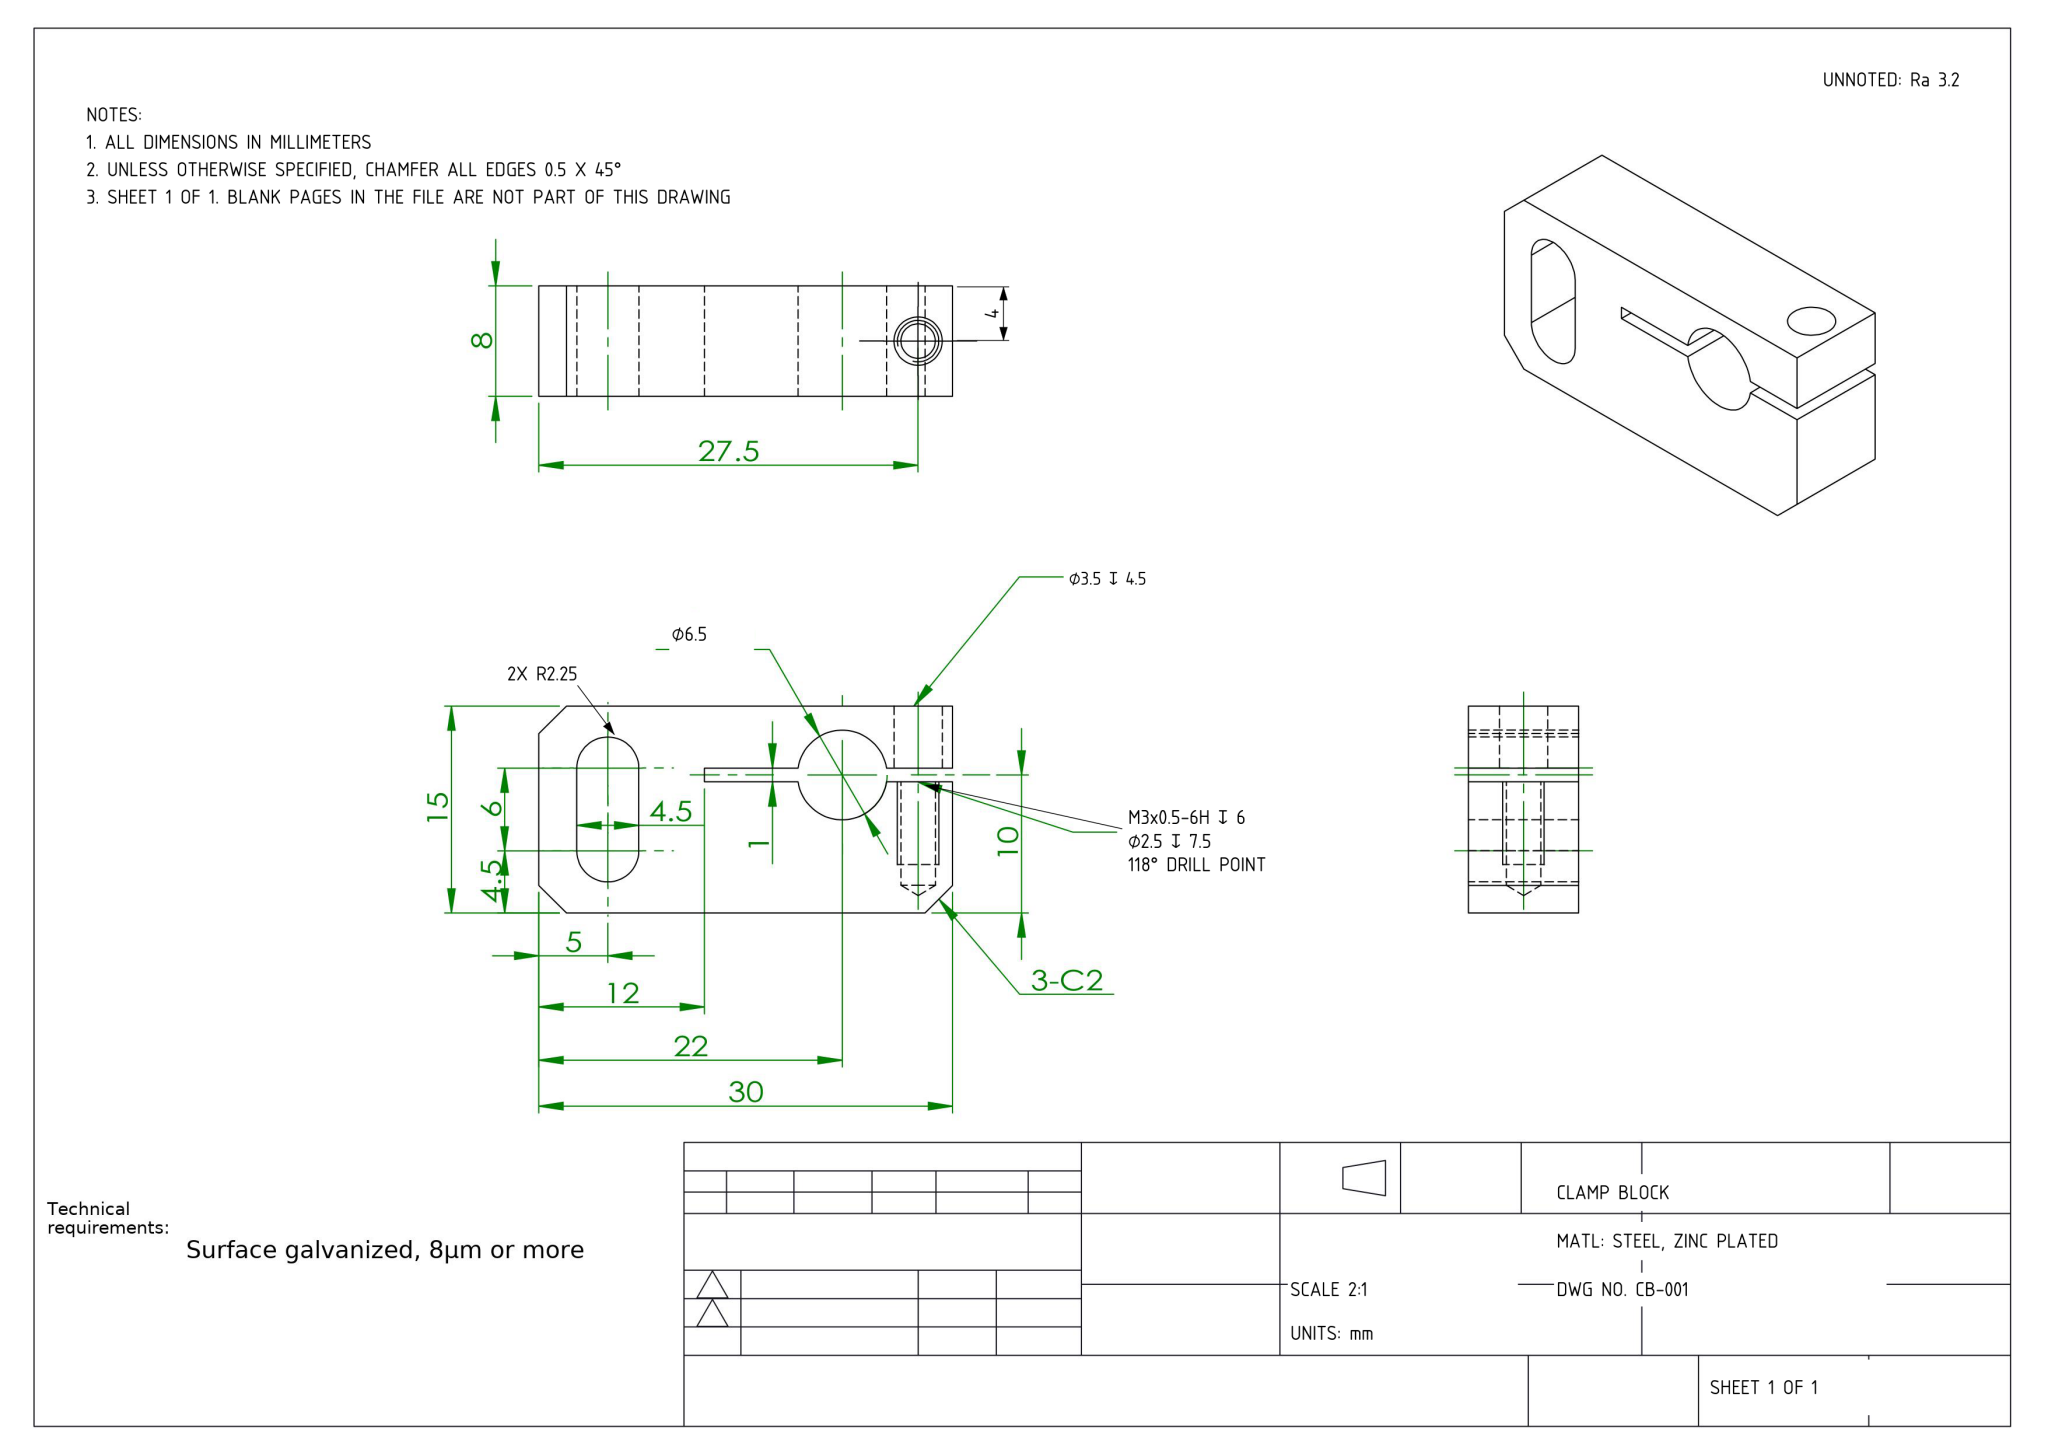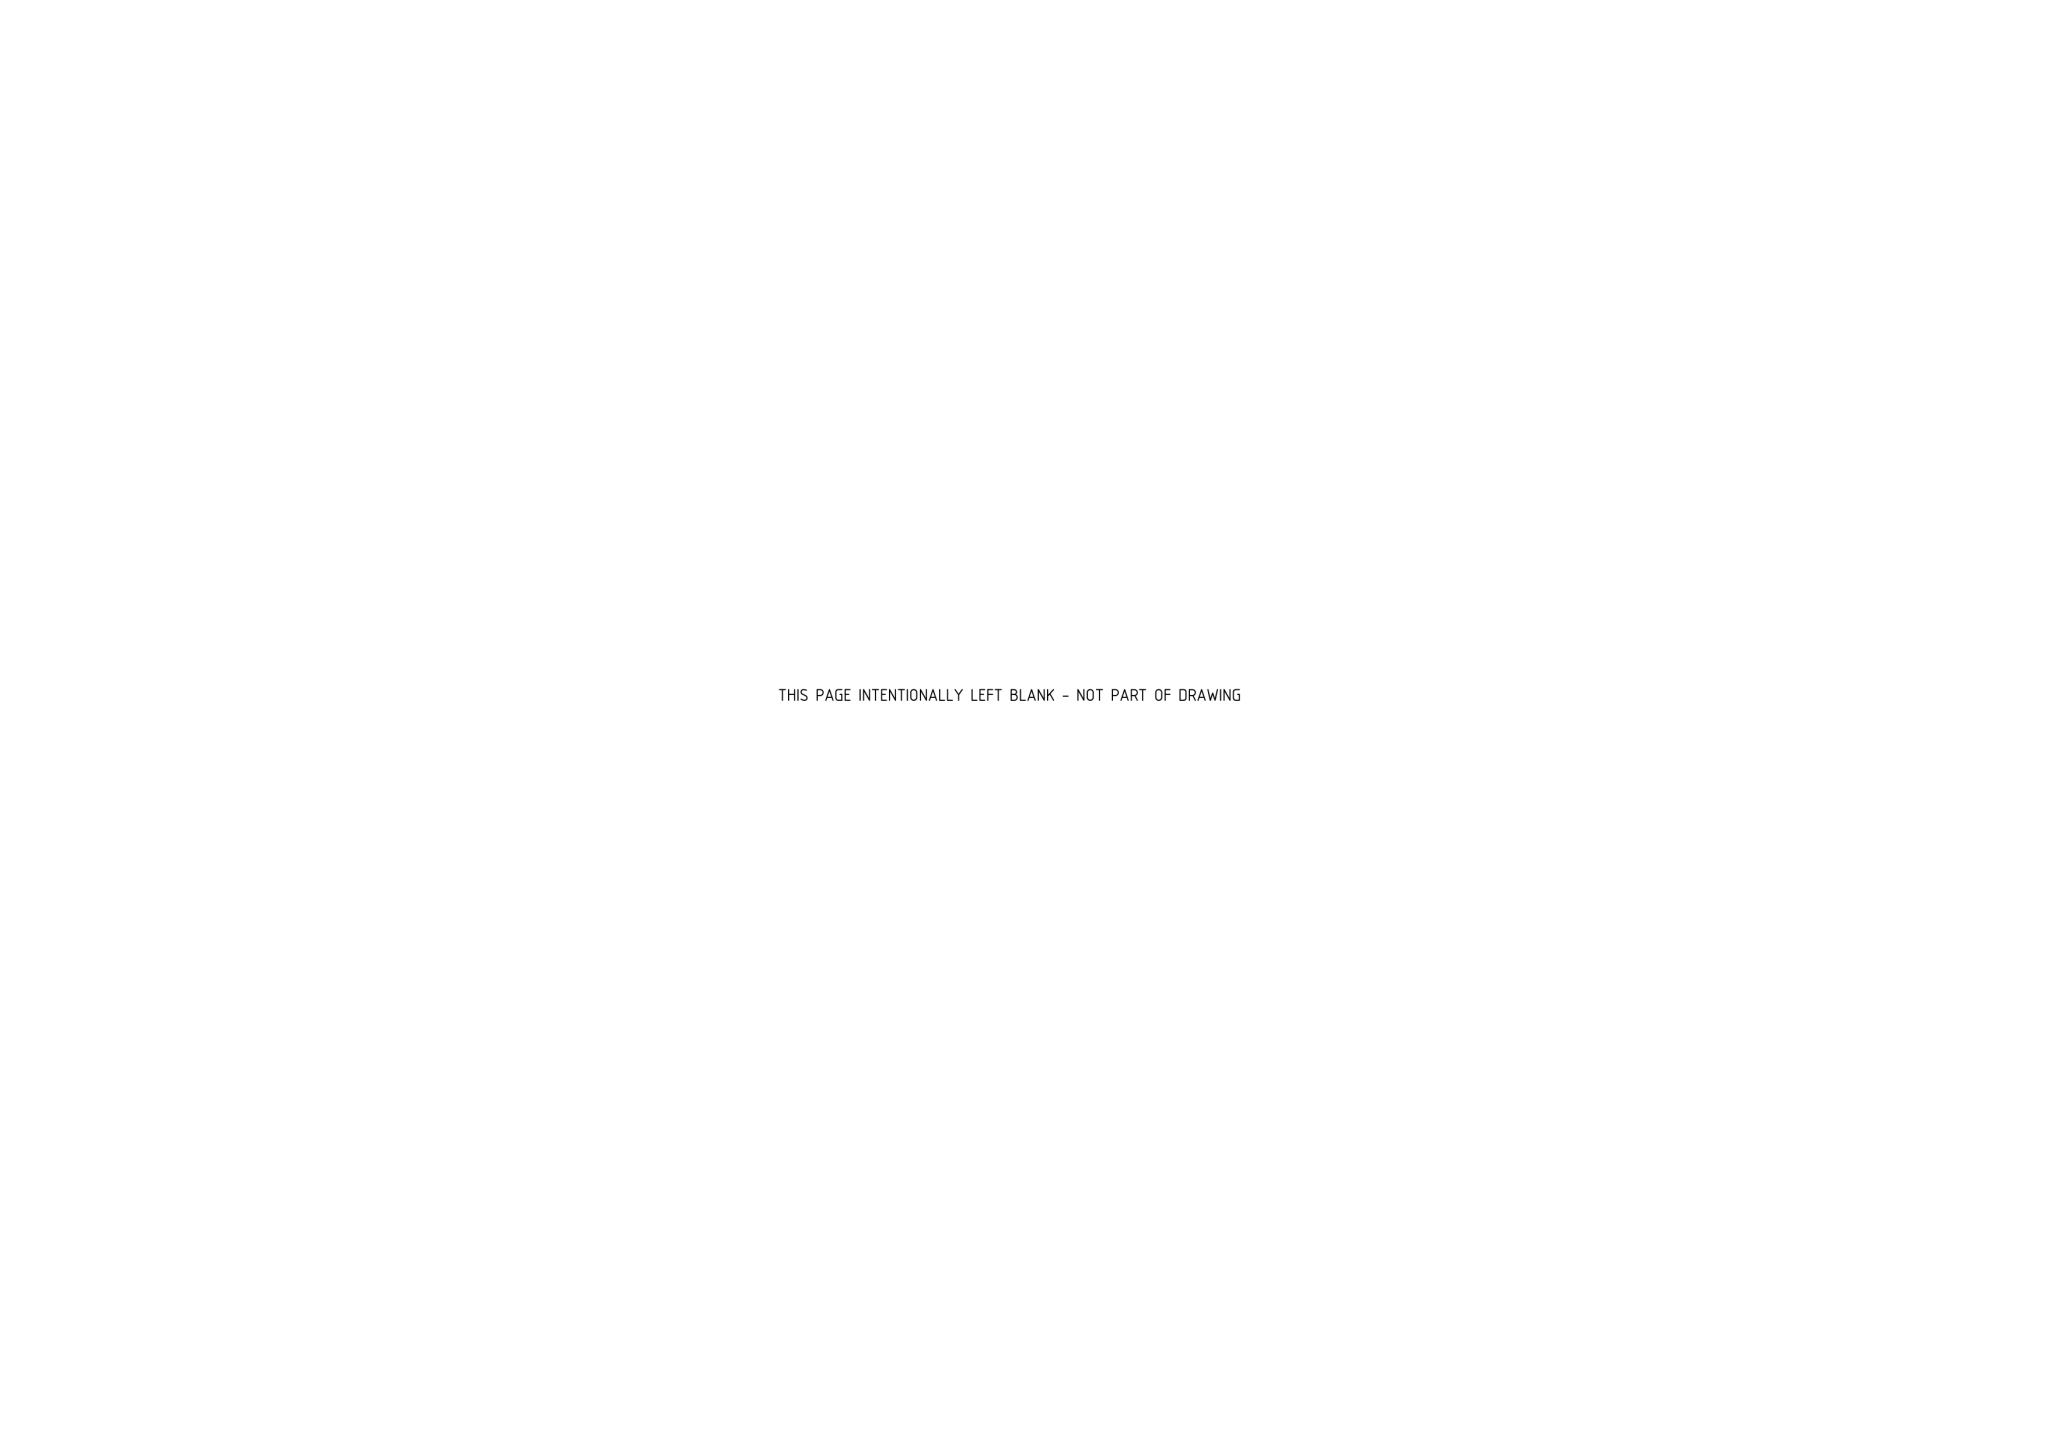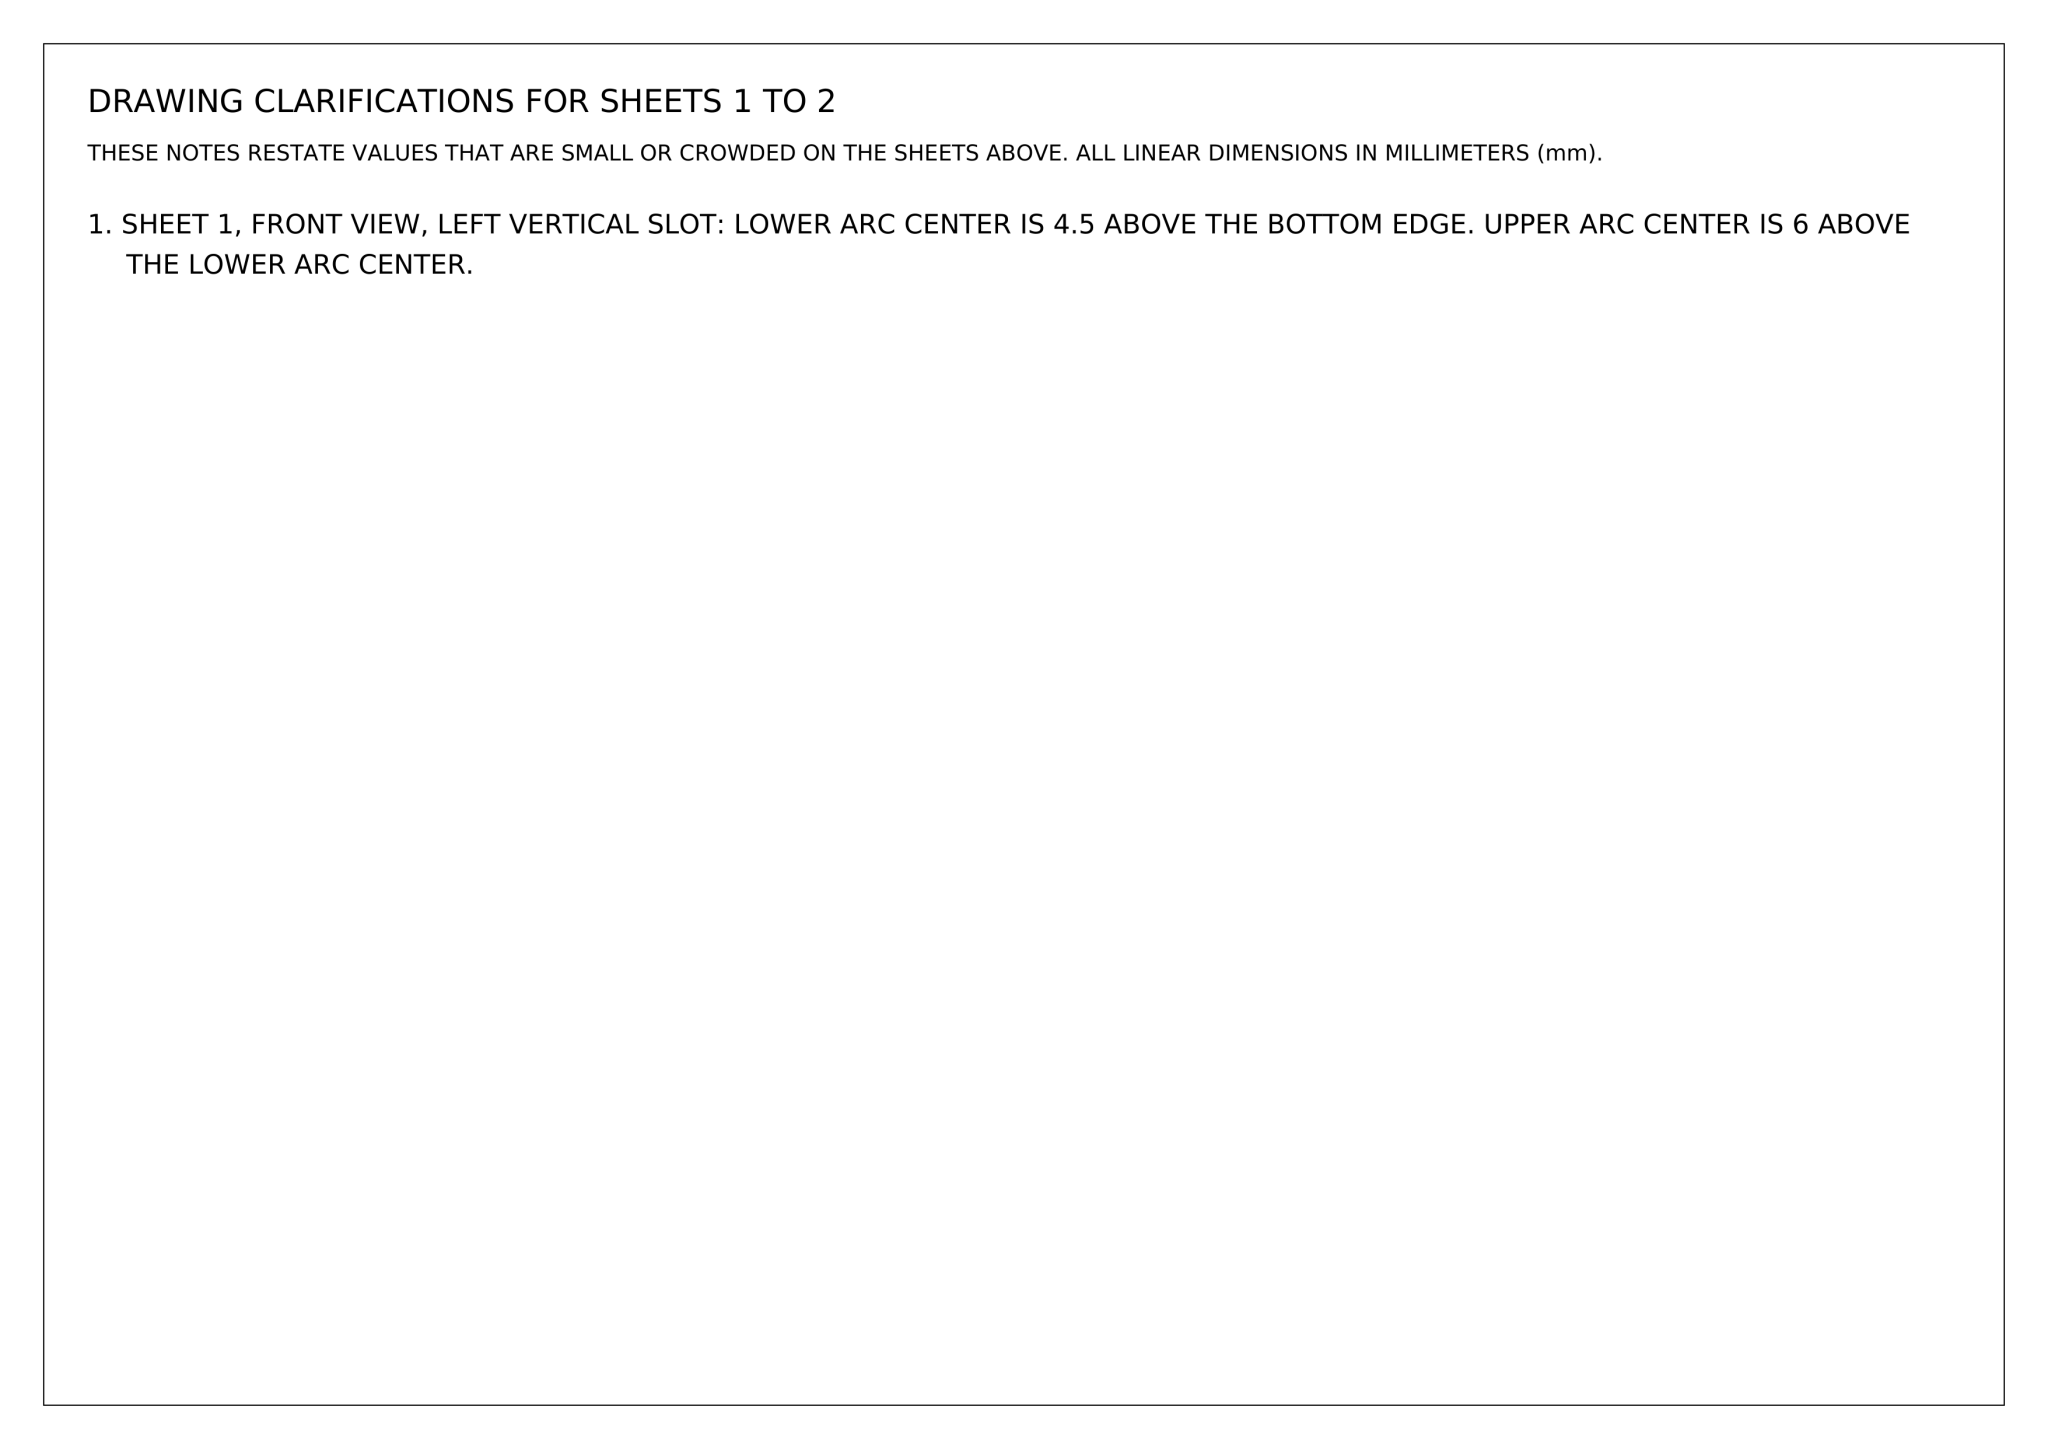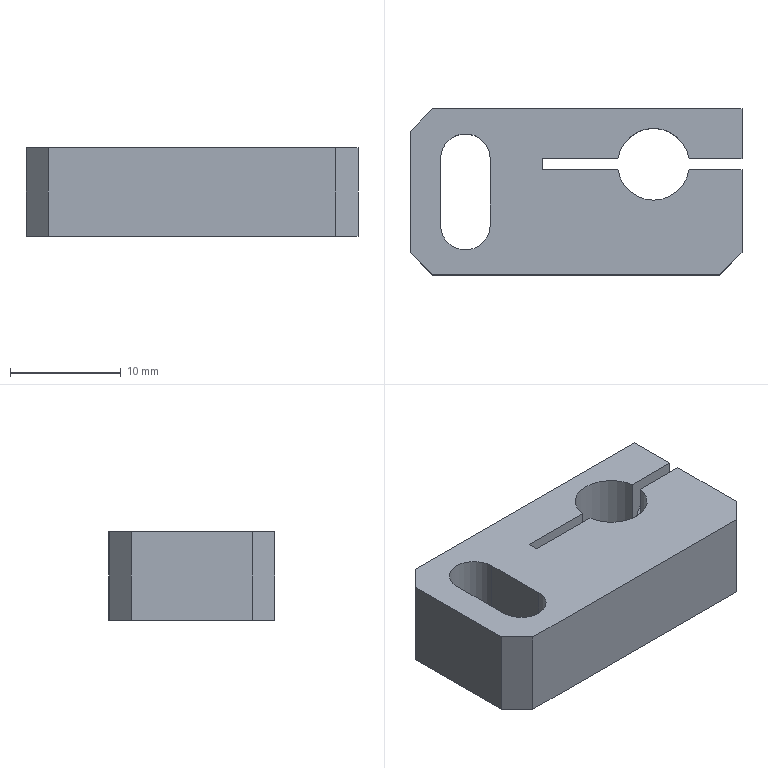Part | NX | mm | 1 solid | 27 faces | box 30 x 15 x 8 mm | volume 2770 mm3 | plane 17 | cylinder 8 | cone 2 | commonest cylinder face diameters 2.5 x2 3.5 x2 4.5 x2 6.5 x2